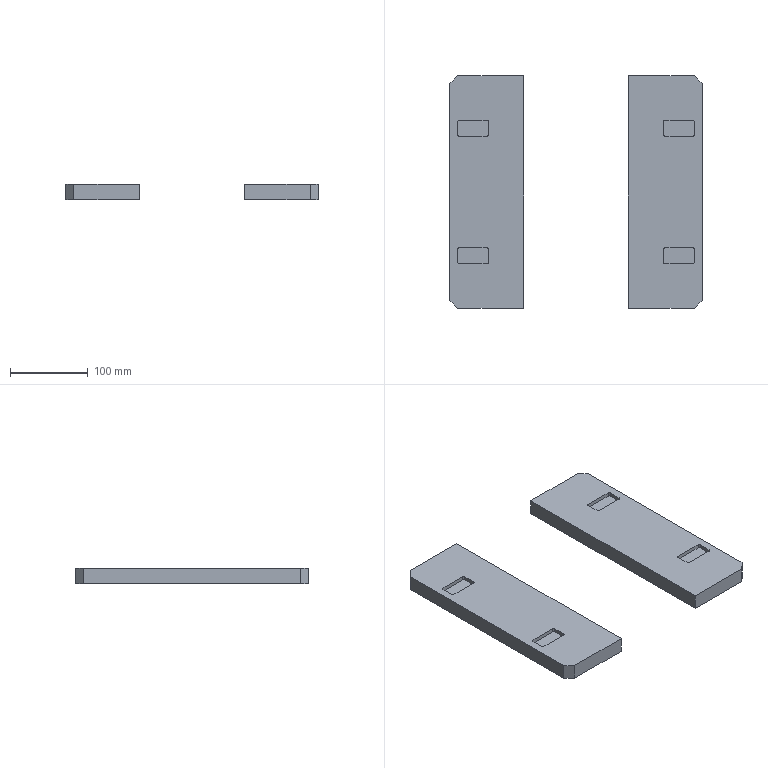Component | SolidWorks | RobotGripperBasePlateAA-1 | 2 solids | 52 faces | box 325 x 300 x 20 mm | volume 1120069 mm3 | plane 36 | cylinder 16 | commonest cylinder face diameters 4 x16 | material Aviation Aluminum-7075
build123d program:
from build123d import *

# Parameters (mm, degrees)
SKETCH1_W           = 325
SKETCH1_H           = 300
BOSS_EXTRUDE1_DEPTH = 20
CUT_EXTRUDE2_DEPTH  = 5
CHAMFER3_SIZE       = 10
CUT_EXTRUDE3_REACH  = 224.05
SKETCH4_W           = 135
SKETCH4_H           = 582.89


with BuildPart() as part:
    # Sketch1 → Boss-Extrude1 (new body)
    with BuildSketch(Plane.XY):
        Rectangle(SKETCH1_W, SKETCH1_H)
    extrude(amount=BOSS_EXTRUDE1_DEPTH)

    # Sketch3 → Cut-Extrude2 (cut)
    with BuildSketch(Plane.XY.offset(20)):
        with BuildLine():
            Line((-114.5, -72), (-150.5, -72))
            ThreePointArc((-150.5, -72), (-151.914, -72.586), (-152.5, -74))
            Line((-152.5, -74), (-152.5, -90))
            ThreePointArc((-152.5, -90), (-151.914, -91.414), (-150.5, -92))
            Line((-150.5, -92), (-114.5, -92))
            ThreePointArc((-114.5, -92), (-113.086, -91.414), (-112.5, -90))
            Line((-112.5, -90), (-112.5, -74))
            ThreePointArc((-112.5, -74), (-113.086, -72.586), (-114.5, -72))
        make_face()
        with BuildLine():
            Line((114.5, -72), (150.5, -72))
            ThreePointArc((150.5, -72), (151.914, -72.586), (152.5, -74))
            Line((152.5, -74), (152.5, -90))
            ThreePointArc((152.5, -90), (151.914, -91.414), (150.5, -92))
            Line((150.5, -92), (114.5, -92))
            ThreePointArc((114.5, -92), (113.086, -91.414), (112.5, -90))
            Line((112.5, -90), (112.5, -74))
            ThreePointArc((112.5, -74), (113.086, -72.586), (114.5, -72))
        make_face()
        with BuildLine():
            Line((-114.5, 92), (-150.5, 92))
            ThreePointArc((-150.5, 92), (-151.914, 91.414), (-152.5, 90))
            Line((-152.5, 90), (-152.5, 74))
            ThreePointArc((-152.5, 74), (-151.914, 72.586), (-150.5, 72))
            Line((-150.5, 72), (-114.5, 72))
            ThreePointArc((-114.5, 72), (-113.086, 72.586), (-112.5, 74))
            Line((-112.5, 74), (-112.5, 90))
            ThreePointArc((-112.5, 90), (-113.086, 91.414), (-114.5, 92))
        make_face()
        with BuildLine():
            Line((150.5, 92), (114.5, 92))
            ThreePointArc((114.5, 92), (113.086, 91.414), (112.5, 90))
            Line((112.5, 90), (112.5, 74))
            ThreePointArc((112.5, 74), (113.086, 72.586), (114.5, 72))
            Line((114.5, 72), (150.5, 72))
            ThreePointArc((150.5, 72), (151.914, 72.586), (152.5, 74))
            Line((152.5, 74), (152.5, 90))
            ThreePointArc((152.5, 90), (151.914, 91.414), (150.5, 92))
        make_face()
    extrude(amount=-CUT_EXTRUDE2_DEPTH, mode=Mode.SUBTRACT)

    # Chamfer3
    chamfer3_edges = [part.edges().sort_by_distance(p)[0] for p in [
        (-162.5, 150, 10),
        (162.5, 150, 10),
        (162.5, -150, 10),
        (-162.5, -150, 10),
    ]]
    chamfer(chamfer3_edges, length=CHAMFER3_SIZE)

    # Sketch4 → Cut-Extrude3 (cut, up to next)
    with BuildSketch(Plane.XY.offset(20), mode=Mode.PRIVATE) as cut_extrude3_sk1:
        Rectangle(SKETCH4_W, SKETCH4_H)
    cut_extrude3_tool1 = extrude(cut_extrude3_sk1.sketch, amount=-CUT_EXTRUDE3_REACH, mode=Mode.PRIVATE) & part.part
    add(cut_extrude3_tool1.solids().sort_by_distance((0, 0, 20))[0], mode=Mode.SUBTRACT)


with BuildPart() as cut_extrude3_piece_1:
    # of the separate pieces the step leaves, piece 1, a body of its own (cut_extrude3_pieces)
    add(part.part.solids().sort_by_distance((152.5, -150, 0))[0])


with BuildPart() as cut_extrude3_piece_2:
    # of the separate pieces the step leaves, piece 2, a body of its own (cut_extrude3_pieces)
    add(part.part.solids().sort_by_distance((-67.5, -150, 0))[0])


solid = Compound([cut_extrude3_piece_1.part, cut_extrude3_piece_2.part])

# Placed as in the assembly
solid = solid.moved(Location((-47.37, -334.626, 477.215), (0, 0, 0)))